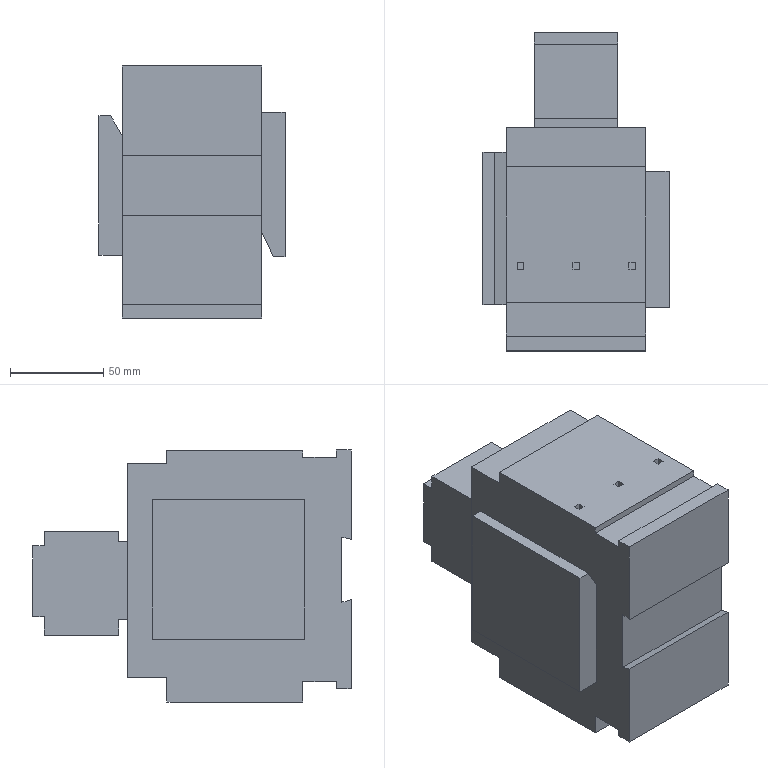Component | SolidWorks | LC1-D40..D65(3-pole)ContactorSchneider-6 | 1 solid | 104 faces | volume 1400649 mm3 | plane 104